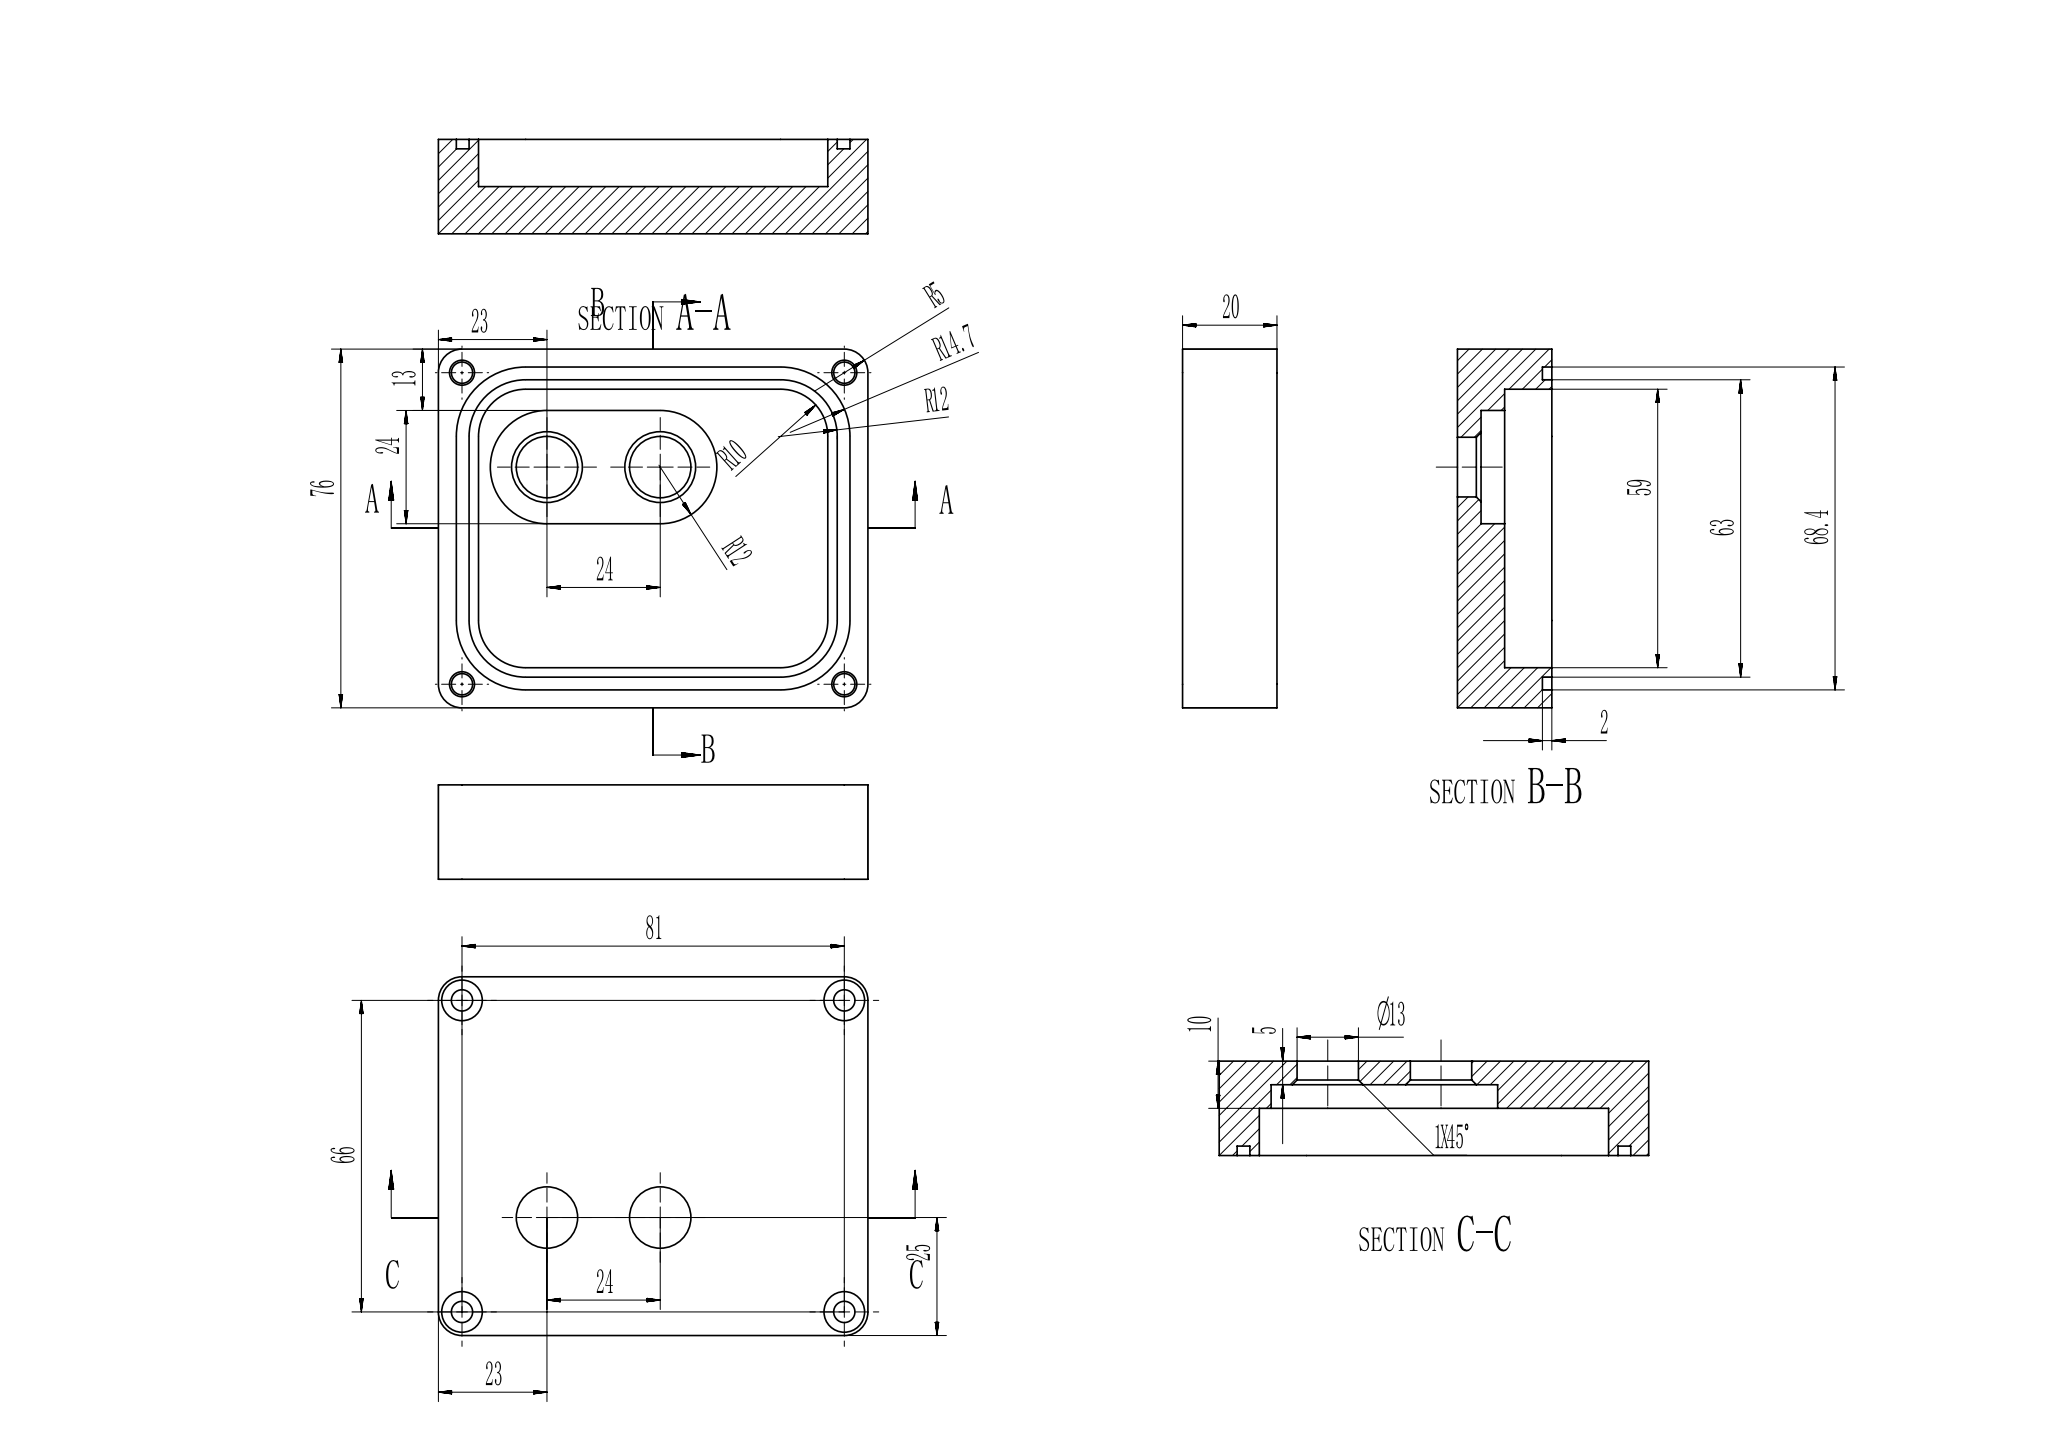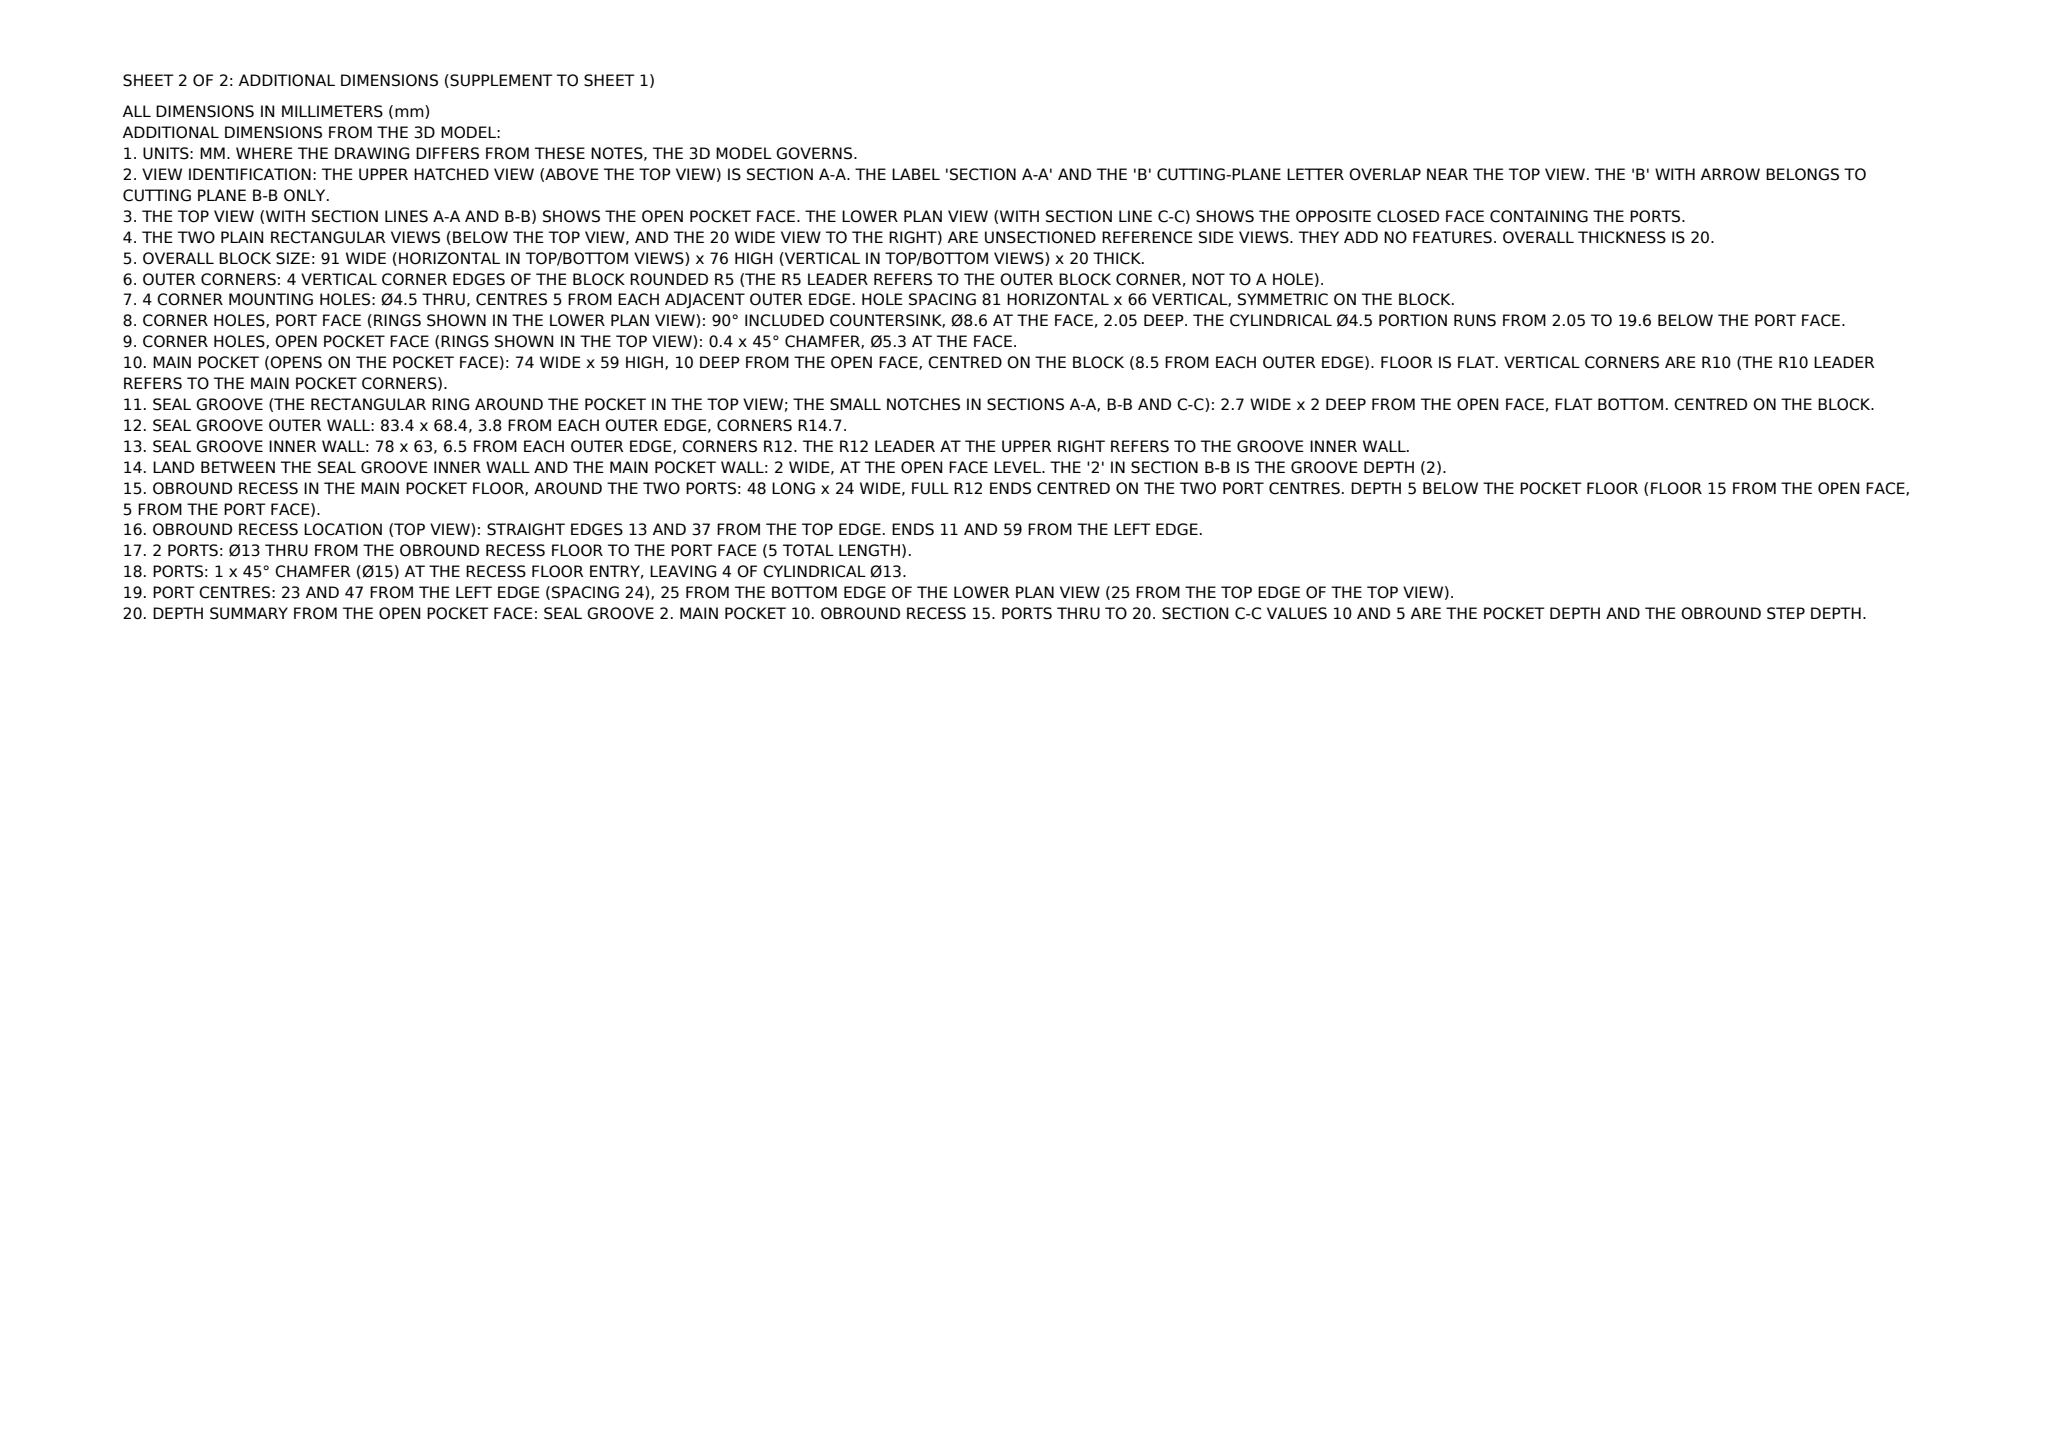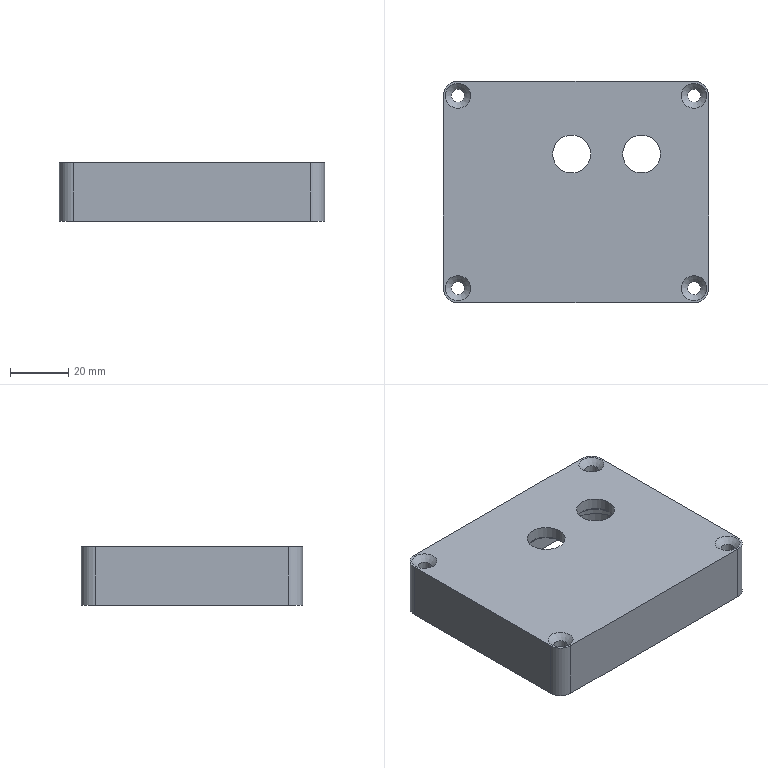Part | NX | mm | 1 solid | 58 faces | box 91 x 76 x 20 mm | volume 85688 mm3 | cylinder 24 | plane 24 | cone 10 | commonest cylinder face diameters 24 x6 10 x4 4.5 x4 20 x4 29.4 x4 13 x2